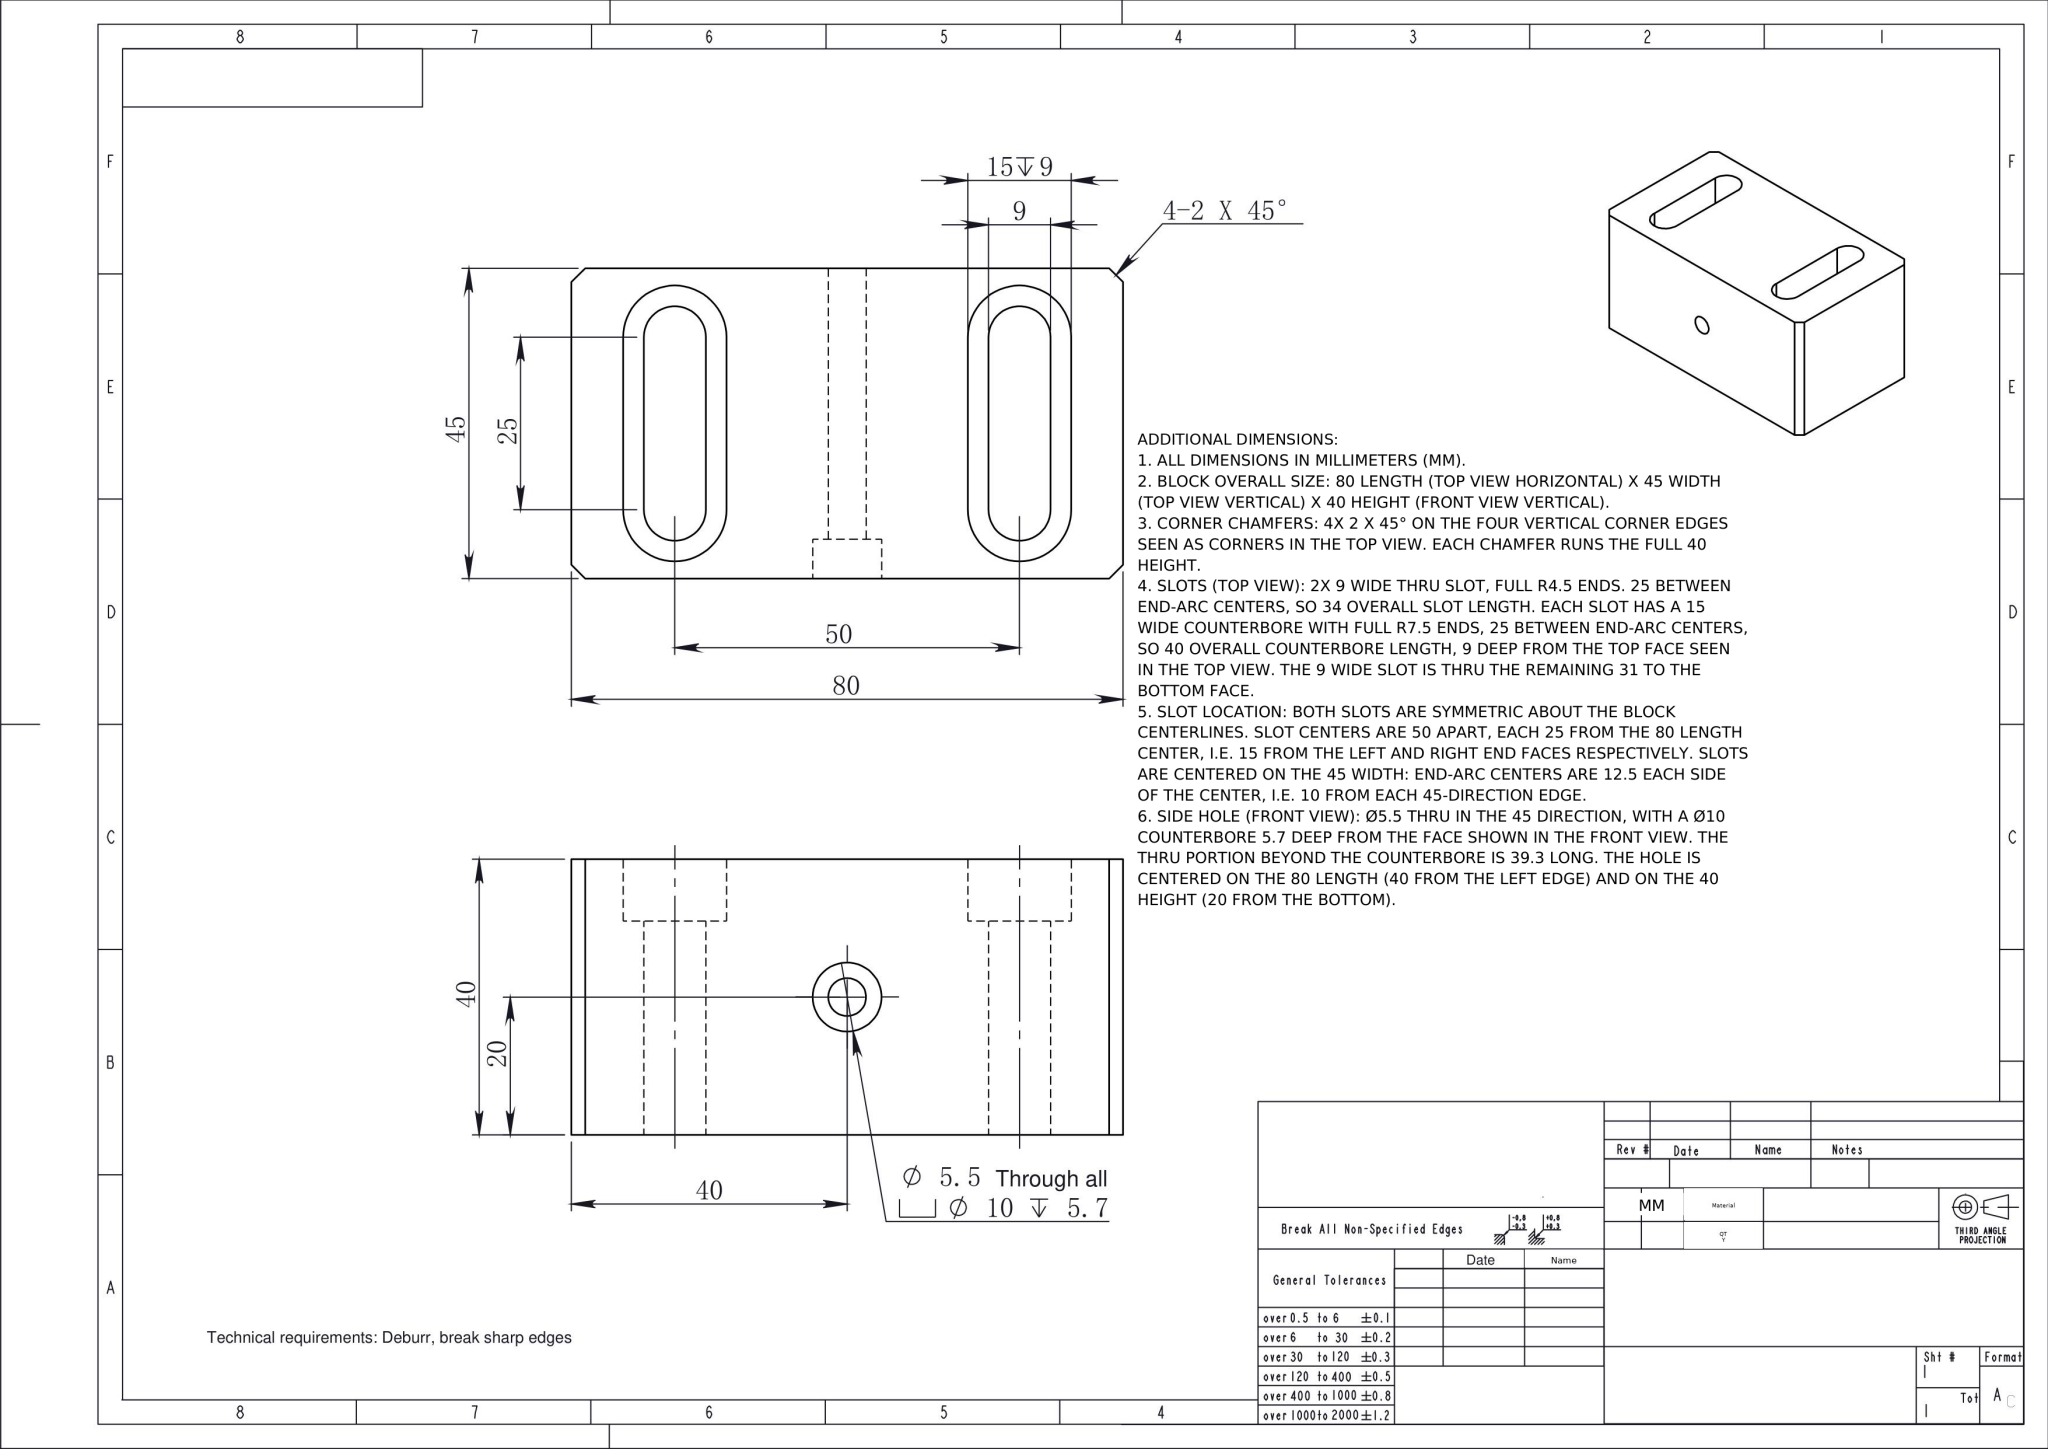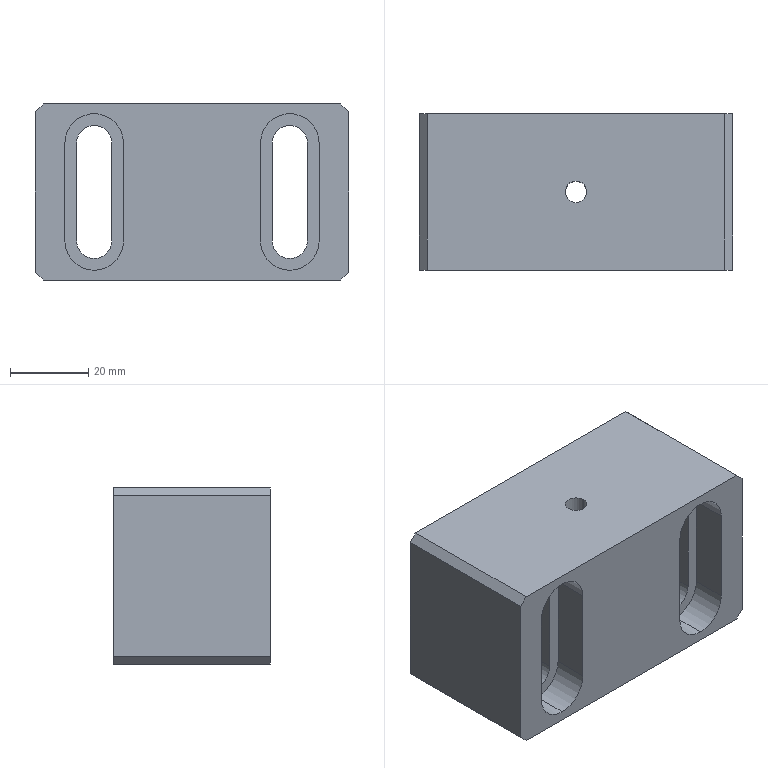Part | NX | mm | 1 solid | 37 faces | box 80 x 40 x 45 mm | volume 114473 mm3 | plane 21 | cylinder 16 | commonest cylinder face diameters 15 x6 9 x6 10 x2 5.5 x2